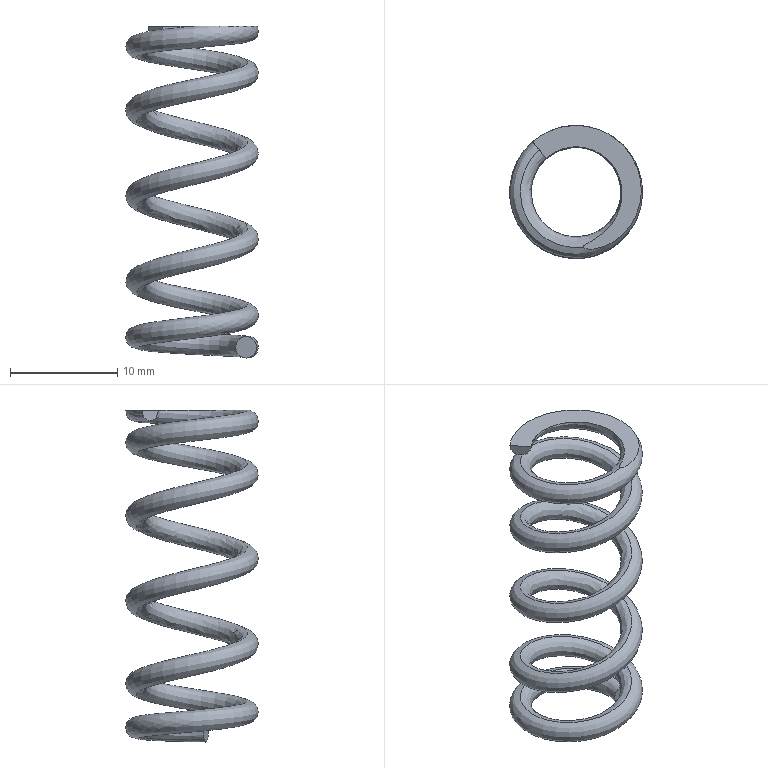Component | SolidWorks | Spring-1 | 1 solid | 5 faces | volume 538 mm3 | plane 3 | spline 2 | material 45